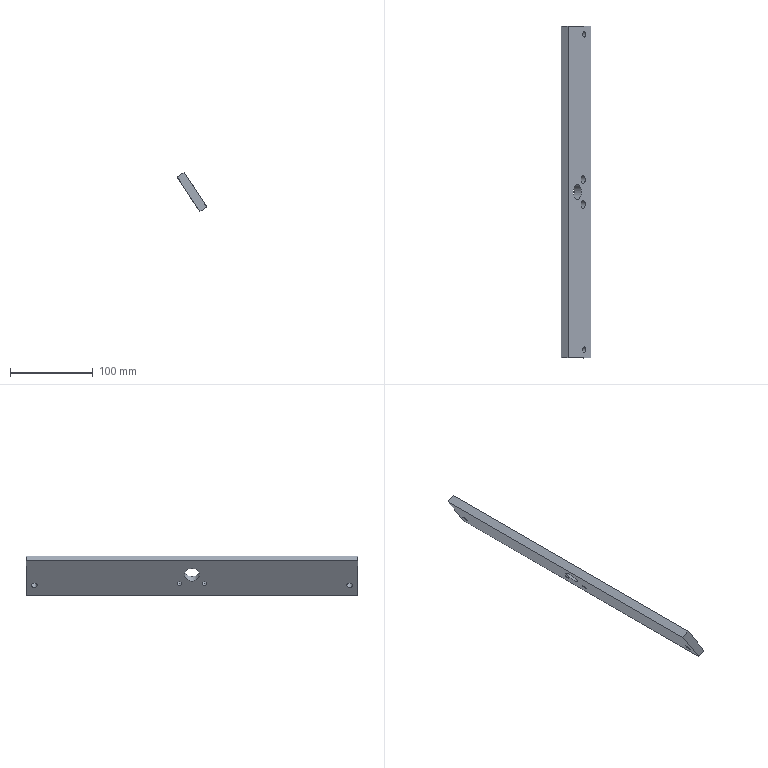Component | SolidWorks | SupportPlate-1 | 1 solid | 22 faces | box 35.72 x 400 x 47.33 mm | volume 195629 mm3 | cylinder 14 | plane 8 | commonest cylinder face diameters 10 x4 5.5 x4 6.8 x4 18 x2
build123d program:
from build123d import *

# Parameters (mm, degrees)
SKETCH1_W                                            = 400
SKETCH1_H                                            = 30
BOSS_EXTRUDE1_DEPTH                                  = 10
M8_TAPPED_HOLE1_D                                    = 6.8
M8_TAPPED_HOLE1_DEPTH                                = 19.75
M8_TAPPED_HOLE1_TIP                                  = 2.043
SKETCH7_W                                            = 400
SKETCH7_H                                            = 10
BOSS_EXTRUDE3_DEPTH                                  = 20
SKETCH9_R                                            = 9
CUT_EXTRUDE2_DEPTH                                   = 204.286
HOLE_SIZE_ACCORDING_TO_THE_TYPE_OF_HEXAG_D           = 5.5
HOLE_SIZE_ACCORDING_TO_THE_TYPE_OF_HEXAG_CBORE_D     = 10
HOLE_SIZE_ACCORDING_TO_THE_TYPE_OF_HEXAG_CBORE_DEPTH = 5.7


with BuildPart() as part:
    # Sketch1 → Boss-Extrude1 (new body)
    with BuildSketch(Plane.XY):
        Rectangle(SKETCH1_W, SKETCH1_H)
    extrude(amount=BOSS_EXTRUDE1_DEPTH)

    # M8 Tapped Hole1
    with Locations(Plane.XY.offset(10)):
        with Locations((-190, 0), (190, 0)):
            Hole(M8_TAPPED_HOLE1_D / 2, depth=M8_TAPPED_HOLE1_DEPTH)
            with Locations((0, 0, -(M8_TAPPED_HOLE1_DEPTH + M8_TAPPED_HOLE1_TIP / 2))):  # 118° drill point
                Cone(0, M8_TAPPED_HOLE1_D / 2, M8_TAPPED_HOLE1_TIP, mode=Mode.SUBTRACT)

    # Sketch7 → Boss-Extrude3 (add)
    with BuildSketch(Plane.XZ.offset(15)):
        with Locations((0, 5)):
            Rectangle(SKETCH7_W, SKETCH7_H)
    extrude(amount=BOSS_EXTRUDE3_DEPTH)

    # Sketch9 → Cut-Extrude2 (cut, through all)
    with BuildSketch(Plane.XY.offset(10)):
        with Locations((0, -15)):
            Circle(SKETCH9_R)
    extrude(amount=-CUT_EXTRUDE2_DEPTH, mode=Mode.SUBTRACT)

    # Hole Size according to the type of hexag (through all)
    with Locations(Plane.XY.offset(10)):
        with Locations((-15, -2.5), (15, -2.5)):
            CounterBoreHole(HOLE_SIZE_ACCORDING_TO_THE_TYPE_OF_HEXAG_D / 2, HOLE_SIZE_ACCORDING_TO_THE_TYPE_OF_HEXAG_CBORE_D / 2, HOLE_SIZE_ACCORDING_TO_THE_TYPE_OF_HEXAG_CBORE_DEPTH)


solid = part.part

# Placed as in the assembly
solid = solid.moved(Location((-212.557, -40.454, -141.988), (0, 56.835, -90)))
STEP:
#1=COLOUR_RGB('',0.7922,0.8196,0.9333);
#2=FILL_AREA_STYLE_COLOUR('',#1);
#3=FILL_AREA_STYLE('',(#2));
#4=SURFACE_STYLE_FILL_AREA(#3);
#5=SURFACE_SIDE_STYLE('',(#4));
#6=SURFACE_STYLE_USAGE(.BOTH.,#5);
#7=PRESENTATION_STYLE_ASSIGNMENT((#6));
#8=CARTESIAN_POINT('',(-8.281,-0.8053,-5.415));
#9=VERTEX_POINT('',#8);
#10=CARTESIAN_POINT('',(-8.281,-1.199,-5.415));
#11=VERTEX_POINT('',#10);
#12=CARTESIAN_POINT('',(-8.281,-1.002,-5.415));
#13=DIRECTION('',(0.8371,-0.,0.5471));
#14=DIRECTION('',(0.,-1.,0.));
#15=AXIS2_PLACEMENT_3D('',#12,#13,#14);
#16=CIRCLE('',#15,0.1969);
#17=EDGE_CURVE('',#9,#11,#16,.T.);
#18=ORIENTED_EDGE('',*,*,#17,.F.);
#19=CARTESIAN_POINT('',(-8.093,-0.8053,-5.292));
#20=VERTEX_POINT('',#19);
#21=CARTESIAN_POINT('',(-8.093,-0.8053,-5.292));
#22=DIRECTION('',(0.8371,-0.,0.5471));
#23=VECTOR('',#22,39.37);
#24=LINE('',#21,#23);
#25=EDGE_CURVE('',#9,#20,#24,.T.);
#26=ORIENTED_EDGE('',*,*,#25,.T.);
#27=CARTESIAN_POINT('',(-8.093,-1.199,-5.292));
#28=VERTEX_POINT('',#27);
#29=CARTESIAN_POINT('',(-8.093,-1.002,-5.292));
#30=DIRECTION('',(0.8371,-0.,0.5471));
#31=DIRECTION('',(0.,-1.,0.));
#32=AXIS2_PLACEMENT_3D('',#29,#30,#31);
#33=CIRCLE('',#32,0.1969);
#34=EDGE_CURVE('',#20,#28,#33,.T.);
#35=ORIENTED_EDGE('',*,*,#34,.T.);
#36=CARTESIAN_POINT('',(-8.093,-1.199,-5.292));
#37=DIRECTION('',(0.8371,-0.,0.5471));
#38=VECTOR('',#37,39.37);
#39=LINE('',#36,#38);
#40=EDGE_CURVE('',#11,#28,#39,.T.);
#41=ORIENTED_EDGE('',*,*,#40,.F.);
#42=EDGE_LOOP('',(#18,#26,#35,#41));
#43=FACE_OUTER_BOUND('',#42,.T.);
#44=CARTESIAN_POINT('',(-8.093,-1.002,-5.292));
#45=DIRECTION('',(0.8371,-0.,0.5471));
#46=DIRECTION('',(0.,-1.,0.));
#47=AXIS2_PLACEMENT_3D('',#44,#45,#46);
#48=CYLINDRICAL_SURFACE('',#47,0.1969);
#49=ADVANCED_FACE('',(#43),#48,.F.);
#50=CARTESIAN_POINT('',(-8.422,-0.8939,-5.508));
#51=VERTEX_POINT('',#50);
#52=CARTESIAN_POINT('',(-8.422,-1.11,-5.508));
#53=VERTEX_POINT('',#52);
#54=CARTESIAN_POINT('',(-8.422,-1.002,-5.508));
#55=DIRECTION('',(0.8371,-0.,0.5471));
#56=DIRECTION('',(0.,-1.,0.));
#57=AXIS2_PLACEMENT_3D('',#54,#55,#56);
#58=CIRCLE('',#57,0.1083);
#59=EDGE_CURVE('',#51,#53,#58,.T.);
#60=ORIENTED_EDGE('',*,*,#59,.F.);
#61=CARTESIAN_POINT('',(-8.281,-0.8939,-5.415));
#62=VERTEX_POINT('',#61);
#63=CARTESIAN_POINT('',(-8.093,-0.8939,-5.292));
#64=DIRECTION('',(0.8371,-0.,0.5471));
#65=VECTOR('',#64,39.37);
#66=LINE('',#63,#65);
#67=EDGE_CURVE('',#51,#62,#66,.T.);
#68=ORIENTED_EDGE('',*,*,#67,.T.);
#69=CARTESIAN_POINT('',(-8.281,-1.11,-5.415));
#70=VERTEX_POINT('',#69);
#71=CARTESIAN_POINT('',(-8.281,-1.002,-5.415));
#72=DIRECTION('',(0.8371,-0.,0.5471));
#73=DIRECTION('',(0.,-1.,0.));
#74=AXIS2_PLACEMENT_3D('',#71,#72,#73);
#75=CIRCLE('',#74,0.1083);
#76=EDGE_CURVE('',#62,#70,#75,.T.);
#77=ORIENTED_EDGE('',*,*,#76,.T.);
#78=CARTESIAN_POINT('',(-8.093,-1.11,-5.292));
#79=DIRECTION('',(0.8371,-0.,0.5471));
#80=VECTOR('',#79,39.37);
#81=LINE('',#78,#80);
#82=EDGE_CURVE('',#53,#70,#81,.T.);
#83=ORIENTED_EDGE('',*,*,#82,.F.);
#84=EDGE_LOOP('',(#60,#68,#77,#83));
#85=FACE_OUTER_BOUND('',#84,.T.);
#86=CARTESIAN_POINT('',(-8.093,-1.002,-5.292));
#87=DIRECTION('',(0.8371,-0.,0.5471));
#88=DIRECTION('',(0.,-1.,0.));
#89=AXIS2_PLACEMENT_3D('',#86,#87,#88);
#90=CYLINDRICAL_SURFACE('',#89,0.1083);
#91=ADVANCED_FACE('',(#85),#90,.F.);
#92=CARTESIAN_POINT('',(-8.281,-1.986,-5.415));
#93=VERTEX_POINT('',#92);
#94=CARTESIAN_POINT('',(-8.281,-2.38,-5.415));
#95=VERTEX_POINT('',#94);
#96=CARTESIAN_POINT('',(-8.281,-2.183,-5.415));
#97=DIRECTION('',(0.8371,-0.,0.5471));
#98=DIRECTION('',(0.,-1.,0.));
#99=AXIS2_PLACEMENT_3D('',#96,#97,#98);
#100=CIRCLE('',#99,0.1969);
#101=EDGE_CURVE('',#93,#95,#100,.T.);
#102=ORIENTED_EDGE('',*,*,#101,.F.);
#103=CARTESIAN_POINT('',(-8.093,-1.986,-5.292));
#104=VERTEX_POINT('',#103);
#105=CARTESIAN_POINT('',(-8.093,-1.986,-5.292));
#106=DIRECTION('',(0.8371,-0.,0.5471));
#107=VECTOR('',#106,39.37);
#108=LINE('',#105,#107);
#109=EDGE_CURVE('',#93,#104,#108,.T.);
#110=ORIENTED_EDGE('',*,*,#109,.T.);
#111=CARTESIAN_POINT('',(-8.093,-2.38,-5.292));
#112=VERTEX_POINT('',#111);
#113=CARTESIAN_POINT('',(-8.093,-2.183,-5.292));
#114=DIRECTION('',(0.8371,-0.,0.5471));
#115=DIRECTION('',(0.,-1.,0.));
#116=AXIS2_PLACEMENT_3D('',#113,#114,#115);
#117=CIRCLE('',#116,0.1969);
#118=EDGE_CURVE('',#104,#112,#117,.T.);
#119=ORIENTED_EDGE('',*,*,#118,.T.);
#120=CARTESIAN_POINT('',(-8.093,-2.38,-5.292));
#121=DIRECTION('',(0.8371,-0.,0.5471));
#122=VECTOR('',#121,39.37);
#123=LINE('',#120,#122);
#124=EDGE_CURVE('',#95,#112,#123,.T.);
#125=ORIENTED_EDGE('',*,*,#124,.F.);
#126=EDGE_LOOP('',(#102,#110,#119,#125));
#127=FACE_OUTER_BOUND('',#126,.T.);
#128=CARTESIAN_POINT('',(-8.093,-2.183,-5.292));
#129=DIRECTION('',(0.8371,-0.,0.5471));
#130=DIRECTION('',(0.,-1.,0.));
#131=AXIS2_PLACEMENT_3D('',#128,#129,#130);
#132=CYLINDRICAL_SURFACE('',#131,0.1969);
#133=ADVANCED_FACE('',(#127),#132,.F.);
#134=CARTESIAN_POINT('',(-8.422,-2.075,-5.508));
#135=VERTEX_POINT('',#134);
#136=CARTESIAN_POINT('',(-8.422,-2.292,-5.508));
#137=VERTEX_POINT('',#136);
#138=CARTESIAN_POINT('',(-8.422,-2.183,-5.508));
#139=DIRECTION('',(0.8371,-0.,0.5471));
#140=DIRECTION('',(0.,-1.,0.));
#141=AXIS2_PLACEMENT_3D('',#138,#139,#140);
#142=CIRCLE('',#141,0.1083);
#143=EDGE_CURVE('',#135,#137,#142,.T.);
#144=ORIENTED_EDGE('',*,*,#143,.F.);
#145=CARTESIAN_POINT('',(-8.281,-2.075,-5.415));
#146=VERTEX_POINT('',#145);
#147=CARTESIAN_POINT('',(-8.093,-2.075,-5.292));
#148=DIRECTION('',(0.8371,-0.,0.5471));
#149=VECTOR('',#148,39.37);
#150=LINE('',#147,#149);
#151=EDGE_CURVE('',#135,#146,#150,.T.);
#152=ORIENTED_EDGE('',*,*,#151,.T.);
#153=CARTESIAN_POINT('',(-8.281,-2.292,-5.415));
#154=VERTEX_POINT('',#153);
#155=CARTESIAN_POINT('',(-8.281,-2.183,-5.415));
#156=DIRECTION('',(0.8371,-0.,0.5471));
#157=DIRECTION('',(0.,-1.,0.));
#158=AXIS2_PLACEMENT_3D('',#155,#156,#157);
#159=CIRCLE('',#158,0.1083);
#160=EDGE_CURVE('',#146,#154,#159,.T.);
#161=ORIENTED_EDGE('',*,*,#160,.T.);
#162=CARTESIAN_POINT('',(-8.093,-2.292,-5.292));
#163=DIRECTION('',(0.8371,-0.,0.5471));
#164=VECTOR('',#163,39.37);
#165=LINE('',#162,#164);
#166=EDGE_CURVE('',#137,#154,#165,.T.);
#167=ORIENTED_EDGE('',*,*,#166,.F.);
#168=EDGE_LOOP('',(#144,#152,#161,#167));
#169=FACE_OUTER_BOUND('',#168,.T.);
#170=CARTESIAN_POINT('',(-8.093,-2.183,-5.292));
#171=DIRECTION('',(0.8371,-0.,0.5471));
#172=DIRECTION('',(0.,-1.,0.));
#173=AXIS2_PLACEMENT_3D('',#170,#171,#172);
#174=CYLINDRICAL_SURFACE('',#173,0.1083);
#175=ADVANCED_FACE('',(#169),#174,.F.);
#176=CARTESIAN_POINT('',(-8.691,-1.238,-5.096));
#177=VERTEX_POINT('',#176);
#178=CARTESIAN_POINT('',(-8.691,-1.947,-5.096));
#179=VERTEX_POINT('',#178);
#180=CARTESIAN_POINT('',(-8.691,-1.593,-5.096));
#181=DIRECTION('',(0.8371,-0.,0.5471));
#182=DIRECTION('',(0.,-1.,0.));
#183=AXIS2_PLACEMENT_3D('',#180,#181,#182);
#184=CIRCLE('',#183,0.3543);
#185=EDGE_CURVE('',#177,#179,#184,.T.);
#186=ORIENTED_EDGE('',*,*,#185,.F.);
#187=CARTESIAN_POINT('',(-8.362,-1.238,-4.88));
#188=VERTEX_POINT('',#187);
#189=CARTESIAN_POINT('',(-8.691,-1.238,-5.096));
#190=DIRECTION('',(0.8371,-0.,0.5471));
#191=VECTOR('',#190,39.37);
#192=LINE('',#189,#191);
#193=EDGE_CURVE('',#177,#188,#192,.T.);
#194=ORIENTED_EDGE('',*,*,#193,.T.);
#195=CARTESIAN_POINT('',(-8.362,-1.947,-4.88));
#196=VERTEX_POINT('',#195);
#197=CARTESIAN_POINT('',(-8.362,-1.593,-4.88));
#198=DIRECTION('',(0.8371,-0.,0.5471));
#199=DIRECTION('',(0.,-1.,0.));
#200=AXIS2_PLACEMENT_3D('',#197,#198,#199);
#201=CIRCLE('',#200,0.3543);
#202=EDGE_CURVE('',#188,#196,#201,.T.);
#203=ORIENTED_EDGE('',*,*,#202,.T.);
#204=CARTESIAN_POINT('',(-8.691,-1.947,-5.096));
#205=DIRECTION('',(0.8371,-0.,0.5471));
#206=VECTOR('',#205,39.37);
#207=LINE('',#204,#206);
#208=EDGE_CURVE('',#179,#196,#207,.T.);
#209=ORIENTED_EDGE('',*,*,#208,.F.);
#210=EDGE_LOOP('',(#186,#194,#203,#209));
#211=FACE_OUTER_BOUND('',#210,.T.);
#212=CARTESIAN_POINT('',(-8.691,-1.593,-5.096));
#213=DIRECTION('',(0.8371,-0.,0.5471));
#214=DIRECTION('',(0.,-1.,0.));
#215=AXIS2_PLACEMENT_3D('',#212,#213,#214);
#216=CYLINDRICAL_SURFACE('',#215,0.3543);
#217=ADVANCED_FACE('',(#211),#216,.F.);
#218=CARTESIAN_POINT('',(-8.368,5.754,-5.59));
#219=VERTEX_POINT('',#218);
#220=CARTESIAN_POINT('',(-8.368,6.021,-5.59));
#221=VERTEX_POINT('',#220);
#222=CARTESIAN_POINT('',(-8.368,5.888,-5.59));
#223=DIRECTION('',(-0.8371,0.,-0.5471));
#224=DIRECTION('',(0.,1.,0.));
#225=AXIS2_PLACEMENT_3D('',#222,#223,#224);
#226=CIRCLE('',#225,0.1339);
#227=EDGE_CURVE('',#219,#221,#226,.T.);
#228=ORIENTED_EDGE('',*,*,#227,.T.);
#229=CARTESIAN_POINT('',(-8.039,6.021,-5.375));
#230=VERTEX_POINT('',#229);
#231=CARTESIAN_POINT('',(-8.039,6.021,-5.375));
#232=DIRECTION('',(0.8371,-0.,0.5471));
#233=VECTOR('',#232,39.37);
#234=LINE('',#231,#233);
#235=EDGE_CURVE('',#221,#230,#234,.T.);
#236=ORIENTED_EDGE('',*,*,#235,.T.);
#237=CARTESIAN_POINT('',(-8.039,5.754,-5.375));
#238=VERTEX_POINT('',#237);
#239=CARTESIAN_POINT('',(-8.039,5.888,-5.375));
#240=DIRECTION('',(0.8371,-0.,0.5471));
#241=DIRECTION('',(0.,-1.,0.));
#242=AXIS2_PLACEMENT_3D('',#239,#240,#241);
#243=CIRCLE('',#242,0.1339);
#244=EDGE_CURVE('',#230,#238,#243,.T.);
#245=ORIENTED_EDGE('',*,*,#244,.T.);
#246=CARTESIAN_POINT('',(-8.039,5.754,-5.375));
#247=DIRECTION('',(0.8371,-0.,0.5471));
#248=VECTOR('',#247,39.37);
#249=LINE('',#246,#248);
#250=EDGE_CURVE('',#219,#238,#249,.T.);
#251=ORIENTED_EDGE('',*,*,#250,.F.);
#252=EDGE_LOOP('',(#228,#236,#245,#251));
#253=FACE_OUTER_BOUND('',#252,.T.);
#254=CARTESIAN_POINT('',(-8.039,5.888,-5.375));
#255=DIRECTION('',(0.8371,-0.,0.5471));
#256=DIRECTION('',(0.,-1.,0.));
#257=AXIS2_PLACEMENT_3D('',#254,#255,#256);
#258=CYLINDRICAL_SURFACE('',#257,0.1339);
#259=ADVANCED_FACE('',(#253),#258,.F.);
#260=CARTESIAN_POINT('',(-8.368,-9.207,-5.59));
#261=VERTEX_POINT('',#260);
#262=CARTESIAN_POINT('',(-8.368,-8.939,-5.59));
#263=VERTEX_POINT('',#262);
#264=CARTESIAN_POINT('',(-8.368,-9.073,-5.59));
#265=DIRECTION('',(-0.8371,0.,-0.5471));
#266=DIRECTION('',(0.,1.,0.));
#267=AXIS2_PLACEMENT_3D('',#264,#265,#266);
#268=CIRCLE('',#267,0.1339);
#269=EDGE_CURVE('',#261,#263,#268,.T.);
#270=ORIENTED_EDGE('',*,*,#269,.T.);
#271=CARTESIAN_POINT('',(-8.039,-8.939,-5.375));
#272=VERTEX_POINT('',#271);
#273=CARTESIAN_POINT('',(-8.039,-8.939,-5.375));
#274=DIRECTION('',(0.8371,-0.,0.5471));
#275=VECTOR('',#274,39.37);
#276=LINE('',#273,#275);
#277=EDGE_CURVE('',#263,#272,#276,.T.);
#278=ORIENTED_EDGE('',*,*,#277,.T.);
#279=CARTESIAN_POINT('',(-8.039,-9.207,-5.375));
#280=VERTEX_POINT('',#279);
#281=CARTESIAN_POINT('',(-8.039,-9.073,-5.375));
#282=DIRECTION('',(0.8371,-0.,0.5471));
#283=DIRECTION('',(0.,-1.,0.));
#284=AXIS2_PLACEMENT_3D('',#281,#282,#283);
#285=CIRCLE('',#284,0.1339);
#286=EDGE_CURVE('',#272,#280,#285,.T.);
#287=ORIENTED_EDGE('',*,*,#286,.T.);
#288=CARTESIAN_POINT('',(-8.039,-9.207,-5.375));
#289=DIRECTION('',(0.8371,-0.,0.5471));
#290=VECTOR('',#289,39.37);
#291=LINE('',#288,#290);
#292=EDGE_CURVE('',#261,#280,#291,.T.);
#293=ORIENTED_EDGE('',*,*,#292,.F.);
#294=EDGE_LOOP('',(#270,#278,#287,#293));
#295=FACE_OUTER_BOUND('',#294,.T.);
#296=CARTESIAN_POINT('',(-8.039,-9.073,-5.375));
#297=DIRECTION('',(0.8371,-0.,0.5471));
#298=DIRECTION('',(0.,-1.,0.));
#299=AXIS2_PLACEMENT_3D('',#296,#297,#298);
#300=CYLINDRICAL_SURFACE('',#299,0.1339);
#301=ADVANCED_FACE('',(#295),#300,.F.);
#302=CARTESIAN_POINT('',(-9.122,-9.467,-4.437));
#303=VERTEX_POINT('',#302);
#304=CARTESIAN_POINT('',(-8.045,-9.467,-6.084));
#305=VERTEX_POINT('',#304);
#306=CARTESIAN_POINT('',(-8.691,-9.467,-5.096));
#307=DIRECTION('',(0.5471,-0.,-0.8371));
#308=VECTOR('',#307,39.37);
#309=LINE('',#306,#308);
#310=EDGE_CURVE('',#303,#305,#309,.T.);
#311=ORIENTED_EDGE('',*,*,#310,.T.);
#312=CARTESIAN_POINT('',(-7.716,-9.467,-5.869));
#313=VERTEX_POINT('',#312);
#314=CARTESIAN_POINT('',(-7.716,-9.467,-5.869));
#315=DIRECTION('',(-0.8371,0.,-0.5471));
#316=VECTOR('',#315,39.37);
#317=LINE('',#314,#316);
#318=EDGE_CURVE('',#313,#305,#317,.T.);
#319=ORIENTED_EDGE('',*,*,#318,.F.);
#320=CARTESIAN_POINT('',(-8.793,-9.467,-4.221));
#321=VERTEX_POINT('',#320);
#322=CARTESIAN_POINT('',(-8.362,-9.467,-4.88));
#323=DIRECTION('',(0.5471,-0.,-0.8371));
#324=VECTOR('',#323,39.37);
#325=LINE('',#322,#324);
#326=EDGE_CURVE('',#321,#313,#325,.T.);
#327=ORIENTED_EDGE('',*,*,#326,.F.);
#328=CARTESIAN_POINT('',(-8.793,-9.467,-4.221));
#329=DIRECTION('',(0.8371,-0.,0.5471));
#330=VECTOR('',#329,39.37);
#331=LINE('',#328,#330);
#332=EDGE_CURVE('',#303,#321,#331,.T.);
#333=ORIENTED_EDGE('',*,*,#332,.F.);
#334=EDGE_LOOP('',(#311,#319,#327,#333));
#335=FACE_OUTER_BOUND('',#334,.T.);
#336=CARTESIAN_POINT('',(-8.362,-9.467,-4.88));
#337=DIRECTION('',(0.,1.,-0.));
#338=DIRECTION('',(0.8371,-0.,0.5471));
#339=AXIS2_PLACEMENT_3D('',#336,#337,#338);
#340=PLANE('',#339);
#341=ADVANCED_FACE('',(#335),#340,.F.);
#342=CARTESIAN_POINT('',(-8.045,6.281,-6.084));
#343=VERTEX_POINT('',#342);
#344=CARTESIAN_POINT('',(-8.045,6.281,-6.084));
#345=DIRECTION('',(0.,1.,-0.));
#346=VECTOR('',#345,39.37);
#347=LINE('',#344,#346);
#348=EDGE_CURVE('',#305,#343,#347,.T.);
#349=ORIENTED_EDGE('',*,*,#348,.T.);
#350=CARTESIAN_POINT('',(-7.716,6.281,-5.869));
#351=VERTEX_POINT('',#350);
#352=CARTESIAN_POINT('',(-7.716,6.281,-5.869));
#353=DIRECTION('',(-0.8371,0.,-0.5471));
#354=VECTOR('',#353,39.37);
#355=LINE('',#352,#354);
#356=EDGE_CURVE('',#351,#343,#355,.T.);
#357=ORIENTED_EDGE('',*,*,#356,.F.);
#358=CARTESIAN_POINT('',(-7.716,6.281,-5.869));
#359=DIRECTION('',(0.,1.,-0.));
#360=VECTOR('',#359,39.37);
#361=LINE('',#358,#360);
#362=EDGE_CURVE('',#313,#351,#361,.T.);
#363=ORIENTED_EDGE('',*,*,#362,.F.);
#364=ORIENTED_EDGE('',*,*,#318,.T.);
#365=EDGE_LOOP('',(#349,#357,#363,#364));
#366=FACE_OUTER_BOUND('',#365,.T.);
#367=CARTESIAN_POINT('',(-7.716,6.281,-5.869));
#368=DIRECTION('',(-0.5471,0.,0.8371));
#369=DIRECTION('',(-0.8371,0.,-0.5471));
#370=AXIS2_PLACEMENT_3D('',#367,#368,#369);
#371=PLANE('',#370);
#372=ADVANCED_FACE('',(#366),#371,.F.);
#373=CARTESIAN_POINT('',(-9.122,6.281,-4.437));
#374=VERTEX_POINT('',#373);
#375=CARTESIAN_POINT('',(-8.691,6.281,-5.096));
#376=DIRECTION('',(-0.5471,0.,0.8371));
#377=VECTOR('',#376,39.37);
#378=LINE('',#375,#377);
#379=EDGE_CURVE('',#343,#374,#378,.T.);
#380=ORIENTED_EDGE('',*,*,#379,.T.);
#381=CARTESIAN_POINT('',(-8.793,6.281,-4.221));
#382=VERTEX_POINT('',#381);
#383=CARTESIAN_POINT('',(-8.793,6.281,-4.221));
#384=DIRECTION('',(-0.8371,0.,-0.5471));
#385=VECTOR('',#384,39.37);
#386=LINE('',#383,#385);
#387=EDGE_CURVE('',#382,#374,#386,.T.);
#388=ORIENTED_EDGE('',*,*,#387,.F.);
#389=CARTESIAN_POINT('',(-8.362,6.281,-4.88));
#390=DIRECTION('',(-0.5471,0.,0.8371));
#391=VECTOR('',#390,39.37);
#392=LINE('',#389,#391);
#393=EDGE_CURVE('',#351,#382,#392,.T.);
#394=ORIENTED_EDGE('',*,*,#393,.F.);
#395=ORIENTED_EDGE('',*,*,#356,.T.);
#396=EDGE_LOOP('',(#380,#388,#394,#395));
#397=FACE_OUTER_BOUND('',#396,.T.);
#398=CARTESIAN_POINT('',(-8.362,6.281,-4.88));
#399=DIRECTION('',(-0.,-1.,0.));
#400=DIRECTION('',(-0.8371,0.,-0.5471));
#401=AXIS2_PLACEMENT_3D('',#398,#399,#400);
#402=PLANE('',#401);
#403=ADVANCED_FACE('',(#397),#402,.F.);
#404=CARTESIAN_POINT('',(-8.093,-1.002,-5.292));
#405=DIRECTION('',(0.8371,-0.,0.5471));
#406=DIRECTION('',(0.,-1.,0.));
#407=AXIS2_PLACEMENT_3D('',#404,#405,#406);
#408=CIRCLE('',#407,0.1969);
#409=EDGE_CURVE('',#28,#20,#408,.T.);
#410=ORIENTED_EDGE('',*,*,#409,.F.);
#411=ORIENTED_EDGE('',*,*,#34,.F.);
#412=EDGE_LOOP('',(#410,#411));
#413=FACE_BOUND('',#412,.T.);
#414=CARTESIAN_POINT('',(-8.093,-2.183,-5.292));
#415=DIRECTION('',(0.8371,-0.,0.5471));
#416=DIRECTION('',(0.,-1.,0.));
#417=AXIS2_PLACEMENT_3D('',#414,#415,#416);
#418=CIRCLE('',#417,0.1969);
#419=EDGE_CURVE('',#112,#104,#418,.T.);
#420=ORIENTED_EDGE('',*,*,#419,.F.);
#421=ORIENTED_EDGE('',*,*,#118,.F.);
#422=EDGE_LOOP('',(#420,#421));
#423=FACE_BOUND('',#422,.T.);
#424=CARTESIAN_POINT('',(-8.362,-1.593,-4.88));
#425=DIRECTION('',(0.8371,-0.,0.5471));
#426=DIRECTION('',(0.,-1.,0.));
#427=AXIS2_PLACEMENT_3D('',#424,#425,#426);
#428=CIRCLE('',#427,0.3543);
#429=EDGE_CURVE('',#196,#188,#428,.T.);
#430=ORIENTED_EDGE('',*,*,#429,.F.);
#431=ORIENTED_EDGE('',*,*,#202,.F.);
#432=EDGE_LOOP('',(#430,#431));
#433=FACE_BOUND('',#432,.T.);
#434=CARTESIAN_POINT('',(-8.039,5.888,-5.375));
#435=DIRECTION('',(0.8371,-0.,0.5471));
#436=DIRECTION('',(0.,-1.,0.));
#437=AXIS2_PLACEMENT_3D('',#434,#435,#436);
#438=CIRCLE('',#437,0.1339);
#439=EDGE_CURVE('',#238,#230,#438,.T.);
#440=ORIENTED_EDGE('',*,*,#439,.F.);
#441=ORIENTED_EDGE('',*,*,#244,.F.);
#442=EDGE_LOOP('',(#440,#441));
#443=FACE_BOUND('',#442,.T.);
#444=CARTESIAN_POINT('',(-8.039,-9.073,-5.375));
#445=DIRECTION('',(0.8371,-0.,0.5471));
#446=DIRECTION('',(0.,-1.,0.));
#447=AXIS2_PLACEMENT_3D('',#444,#445,#446);
#448=CIRCLE('',#447,0.1339);
#449=EDGE_CURVE('',#280,#272,#448,.T.);
#450=ORIENTED_EDGE('',*,*,#449,.F.);
#451=ORIENTED_EDGE('',*,*,#286,.F.);
#452=EDGE_LOOP('',(#450,#451));
#453=FACE_BOUND('',#452,.T.);
#454=ORIENTED_EDGE('',*,*,#326,.T.);
#455=ORIENTED_EDGE('',*,*,#362,.T.);
#456=ORIENTED_EDGE('',*,*,#393,.T.);
#457=CARTESIAN_POINT('',(-8.793,6.281,-4.221));
#458=DIRECTION('',(0.,1.,-0.));
#459=VECTOR('',#458,39.37);
#460=LINE('',#457,#459);
#461=EDGE_CURVE('',#321,#382,#460,.T.);
#462=ORIENTED_EDGE('',*,*,#461,.F.);
#463=EDGE_LOOP('',(#454,#455,#456,#462));
#464=FACE_OUTER_BOUND('',#463,.T.);
#465=CARTESIAN_POINT('',(-8.039,-1.593,-5.375));
#466=DIRECTION('',(-0.8371,0.,-0.5471));
#467=DIRECTION('',(0.,1.,-0.));
#468=AXIS2_PLACEMENT_3D('',#465,#466,#467);
#469=PLANE('',#468);
#470=ADVANCED_FACE('',(#413,#423,#433,#443,#453,#464),#469,.F.);
#471=CARTESIAN_POINT('',(-8.422,-1.002,-5.508));
#472=DIRECTION('',(0.8371,-0.,0.5471));
#473=DIRECTION('',(0.,-1.,0.));
#474=AXIS2_PLACEMENT_3D('',#471,#472,#473);
#475=CIRCLE('',#474,0.1083);
#476=EDGE_CURVE('',#53,#51,#475,.T.);
#477=ORIENTED_EDGE('',*,*,#476,.T.);
#478=ORIENTED_EDGE('',*,*,#59,.T.);
#479=EDGE_LOOP('',(#477,#478));
#480=FACE_BOUND('',#479,.T.);
#481=CARTESIAN_POINT('',(-8.422,-2.183,-5.508));
#482=DIRECTION('',(0.8371,-0.,0.5471));
#483=DIRECTION('',(0.,-1.,0.));
#484=AXIS2_PLACEMENT_3D('',#481,#482,#483);
#485=CIRCLE('',#484,0.1083);
#486=EDGE_CURVE('',#137,#135,#485,.T.);
#487=ORIENTED_EDGE('',*,*,#486,.T.);
#488=ORIENTED_EDGE('',*,*,#143,.T.);
#489=EDGE_LOOP('',(#487,#488));
#490=FACE_BOUND('',#489,.T.);
#491=CARTESIAN_POINT('',(-8.691,-1.593,-5.096));
#492=DIRECTION('',(0.8371,-0.,0.5471));
#493=DIRECTION('',(0.,-1.,0.));
#494=AXIS2_PLACEMENT_3D('',#491,#492,#493);
#495=CIRCLE('',#494,0.3543);
#496=EDGE_CURVE('',#179,#177,#495,.T.);
#497=ORIENTED_EDGE('',*,*,#496,.T.);
#498=ORIENTED_EDGE('',*,*,#185,.T.);
#499=EDGE_LOOP('',(#497,#498));
#500=FACE_BOUND('',#499,.T.);
#501=ORIENTED_EDGE('',*,*,#227,.F.);
#502=CARTESIAN_POINT('',(-8.368,5.888,-5.59));
#503=DIRECTION('',(-0.8371,0.,-0.5471));
#504=DIRECTION('',(0.,1.,0.));
#505=AXIS2_PLACEMENT_3D('',#502,#503,#504);
#506=CIRCLE('',#505,0.1339);
#507=EDGE_CURVE('',#221,#219,#506,.T.);
#508=ORIENTED_EDGE('',*,*,#507,.F.);
#509=EDGE_LOOP('',(#501,#508));
#510=FACE_BOUND('',#509,.T.);
#511=ORIENTED_EDGE('',*,*,#269,.F.);
#512=CARTESIAN_POINT('',(-8.368,-9.073,-5.59));
#513=DIRECTION('',(-0.8371,0.,-0.5471));
#514=DIRECTION('',(0.,1.,0.));
#515=AXIS2_PLACEMENT_3D('',#512,#513,#514);
#516=CIRCLE('',#515,0.1339);
#517=EDGE_CURVE('',#263,#261,#516,.T.);
#518=ORIENTED_EDGE('',*,*,#517,.F.);
#519=EDGE_LOOP('',(#511,#518));
#520=FACE_BOUND('',#519,.T.);
#521=ORIENTED_EDGE('',*,*,#310,.F.);
#522=CARTESIAN_POINT('',(-9.122,6.281,-4.437));
#523=DIRECTION('',(-0.,-1.,0.));
#524=VECTOR('',#523,39.37);
#525=LINE('',#522,#524);
#526=EDGE_CURVE('',#374,#303,#525,.T.);
#527=ORIENTED_EDGE('',*,*,#526,.F.);
#528=ORIENTED_EDGE('',*,*,#379,.F.);
#529=ORIENTED_EDGE('',*,*,#348,.F.);
#530=EDGE_LOOP('',(#521,#527,#528,#529));
#531=FACE_OUTER_BOUND('',#530,.T.);
#532=CARTESIAN_POINT('',(-8.368,-1.593,-5.59));
#533=DIRECTION('',(-0.8371,0.,-0.5471));
#534=DIRECTION('',(0.,1.,-0.));
#535=AXIS2_PLACEMENT_3D('',#532,#533,#534);
#536=PLANE('',#535);
#537=ADVANCED_FACE('',(#480,#490,#500,#510,#520,#531),#536,.T.);
#538=ORIENTED_EDGE('',*,*,#277,.F.);
#539=ORIENTED_EDGE('',*,*,#517,.T.);
#540=ORIENTED_EDGE('',*,*,#292,.T.);
#541=ORIENTED_EDGE('',*,*,#449,.T.);
#542=EDGE_LOOP('',(#538,#539,#540,#541));
#543=FACE_OUTER_BOUND('',#542,.T.);
#544=CARTESIAN_POINT('',(-8.039,-9.073,-5.375));
#545=DIRECTION('',(0.8371,-0.,0.5471));
#546=DIRECTION('',(0.,-1.,0.));
#547=AXIS2_PLACEMENT_3D('',#544,#545,#546);
#548=CYLINDRICAL_SURFACE('',#547,0.1339);
#549=ADVANCED_FACE('',(#543),#548,.F.);
#550=ORIENTED_EDGE('',*,*,#235,.F.);
#551=ORIENTED_EDGE('',*,*,#507,.T.);
#552=ORIENTED_EDGE('',*,*,#250,.T.);
#553=ORIENTED_EDGE('',*,*,#439,.T.);
#554=EDGE_LOOP('',(#550,#551,#552,#553));
#555=FACE_OUTER_BOUND('',#554,.T.);
#556=CARTESIAN_POINT('',(-8.039,5.888,-5.375));
#557=DIRECTION('',(0.8371,-0.,0.5471));
#558=DIRECTION('',(0.,-1.,0.));
#559=AXIS2_PLACEMENT_3D('',#556,#557,#558);
#560=CYLINDRICAL_SURFACE('',#559,0.1339);
#561=ADVANCED_FACE('',(#555),#560,.F.);
#562=ORIENTED_EDGE('',*,*,#387,.T.);
#563=ORIENTED_EDGE('',*,*,#526,.T.);
#564=ORIENTED_EDGE('',*,*,#332,.T.);
#565=ORIENTED_EDGE('',*,*,#461,.T.);
#566=EDGE_LOOP('',(#562,#563,#564,#565));
#567=FACE_OUTER_BOUND('',#566,.T.);
#568=CARTESIAN_POINT('',(-9.122,-1.593,-4.437));
#569=DIRECTION('',(-0.5471,0.,0.8371));
#570=DIRECTION('',(-0.8371,0.,-0.5471));
#571=AXIS2_PLACEMENT_3D('',#568,#569,#570);
#572=PLANE('',#571);
#573=ADVANCED_FACE('',(#567),#572,.T.);
#574=ORIENTED_EDGE('',*,*,#193,.F.);
#575=ORIENTED_EDGE('',*,*,#496,.F.);
#576=ORIENTED_EDGE('',*,*,#208,.T.);
#577=ORIENTED_EDGE('',*,*,#429,.T.);
#578=EDGE_LOOP('',(#574,#575,#576,#577));
#579=FACE_OUTER_BOUND('',#578,.T.);
#580=CARTESIAN_POINT('',(-8.691,-1.593,-5.096));
#581=DIRECTION('',(0.8371,-0.,0.5471));
#582=DIRECTION('',(0.,-1.,0.));
#583=AXIS2_PLACEMENT_3D('',#580,#581,#582);
#584=CYLINDRICAL_SURFACE('',#583,0.3543);
#585=ADVANCED_FACE('',(#579),#584,.F.);
#586=ORIENTED_EDGE('',*,*,#151,.F.);
#587=ORIENTED_EDGE('',*,*,#486,.F.);
#588=ORIENTED_EDGE('',*,*,#166,.T.);
#589=CARTESIAN_POINT('',(-8.281,-2.183,-5.415));
#590=DIRECTION('',(0.8371,-0.,0.5471));
#591=DIRECTION('',(0.,-1.,0.));
#592=AXIS2_PLACEMENT_3D('',#589,#590,#591);
#593=CIRCLE('',#592,0.1083);
#594=EDGE_CURVE('',#154,#146,#593,.T.);
#595=ORIENTED_EDGE('',*,*,#594,.T.);
#596=EDGE_LOOP('',(#586,#587,#588,#595));
#597=FACE_OUTER_BOUND('',#596,.T.);
#598=CARTESIAN_POINT('',(-8.093,-2.183,-5.292));
#599=DIRECTION('',(0.8371,-0.,0.5471));
#600=DIRECTION('',(0.,-1.,0.));
#601=AXIS2_PLACEMENT_3D('',#598,#599,#600);
#602=CYLINDRICAL_SURFACE('',#601,0.1083);
#603=ADVANCED_FACE('',(#597),#602,.F.);
#604=ORIENTED_EDGE('',*,*,#594,.F.);
#605=ORIENTED_EDGE('',*,*,#160,.F.);
#606=EDGE_LOOP('',(#604,#605));
#607=FACE_BOUND('',#606,.T.);
#608=CARTESIAN_POINT('',(-8.281,-2.183,-5.415));
#609=DIRECTION('',(0.8371,-0.,0.5471));
#610=DIRECTION('',(0.,-1.,0.));
#611=AXIS2_PLACEMENT_3D('',#608,#609,#610);
#612=CIRCLE('',#611,0.1969);
#613=EDGE_CURVE('',#95,#93,#612,.T.);
#614=ORIENTED_EDGE('',*,*,#613,.T.);
#615=ORIENTED_EDGE('',*,*,#101,.T.);
#616=EDGE_LOOP('',(#614,#615));
#617=FACE_OUTER_BOUND('',#616,.T.);
#618=CARTESIAN_POINT('',(-8.281,-2.292,-5.415));
#619=DIRECTION('',(-0.8371,0.,-0.5471));
#620=DIRECTION('',(0.,1.,-0.));
#621=AXIS2_PLACEMENT_3D('',#618,#619,#620);
#622=PLANE('',#621);
#623=ADVANCED_FACE('',(#607,#617),#622,.F.);
#624=ORIENTED_EDGE('',*,*,#109,.F.);
#625=ORIENTED_EDGE('',*,*,#613,.F.);
#626=ORIENTED_EDGE('',*,*,#124,.T.);
#627=ORIENTED_EDGE('',*,*,#419,.T.);
#628=EDGE_LOOP('',(#624,#625,#626,#627));
#629=FACE_OUTER_BOUND('',#628,.T.);
#630=CARTESIAN_POINT('',(-8.093,-2.183,-5.292));
#631=DIRECTION('',(0.8371,-0.,0.5471));
#632=DIRECTION('',(0.,-1.,0.));
#633=AXIS2_PLACEMENT_3D('',#630,#631,#632);
#634=CYLINDRICAL_SURFACE('',#633,0.1969);
#635=ADVANCED_FACE('',(#629),#634,.F.);
#636=ORIENTED_EDGE('',*,*,#67,.F.);
#637=ORIENTED_EDGE('',*,*,#476,.F.);
#638=ORIENTED_EDGE('',*,*,#82,.T.);
#639=CARTESIAN_POINT('',(-8.281,-1.002,-5.415));
#640=DIRECTION('',(0.8371,-0.,0.5471));
#641=DIRECTION('',(0.,-1.,0.));
#642=AXIS2_PLACEMENT_3D('',#639,#640,#641);
#643=CIRCLE('',#642,0.1083);
#644=EDGE_CURVE('',#70,#62,#643,.T.);
#645=ORIENTED_EDGE('',*,*,#644,.T.);
#646=EDGE_LOOP('',(#636,#637,#638,#645));
#647=FACE_OUTER_BOUND('',#646,.T.);
#648=CARTESIAN_POINT('',(-8.093,-1.002,-5.292));
#649=DIRECTION('',(0.8371,-0.,0.5471));
#650=DIRECTION('',(0.,-1.,0.));
#651=AXIS2_PLACEMENT_3D('',#648,#649,#650);
#652=CYLINDRICAL_SURFACE('',#651,0.1083);
#653=ADVANCED_FACE('',(#647),#652,.F.);
#654=ORIENTED_EDGE('',*,*,#644,.F.);
#655=ORIENTED_EDGE('',*,*,#76,.F.);
#656=EDGE_LOOP('',(#654,#655));
#657=FACE_BOUND('',#656,.T.);
#658=CARTESIAN_POINT('',(-8.281,-1.002,-5.415));
#659=DIRECTION('',(0.8371,-0.,0.5471));
#660=DIRECTION('',(0.,-1.,0.));
#661=AXIS2_PLACEMENT_3D('',#658,#659,#660);
#662=CIRCLE('',#661,0.1969);
#663=EDGE_CURVE('',#11,#9,#662,.T.);
#664=ORIENTED_EDGE('',*,*,#663,.T.);
#665=ORIENTED_EDGE('',*,*,#17,.T.);
#666=EDGE_LOOP('',(#664,#665));
#667=FACE_OUTER_BOUND('',#666,.T.);
#668=CARTESIAN_POINT('',(-8.281,-1.11,-5.415));
#669=DIRECTION('',(-0.8371,0.,-0.5471));
#670=DIRECTION('',(0.,1.,-0.));
#671=AXIS2_PLACEMENT_3D('',#668,#669,#670);
#672=PLANE('',#671);
#673=ADVANCED_FACE('',(#657,#667),#672,.F.);
#674=ORIENTED_EDGE('',*,*,#25,.F.);
#675=ORIENTED_EDGE('',*,*,#663,.F.);
#676=ORIENTED_EDGE('',*,*,#40,.T.);
#677=ORIENTED_EDGE('',*,*,#409,.T.);
#678=EDGE_LOOP('',(#674,#675,#676,#677));
#679=FACE_OUTER_BOUND('',#678,.T.);
#680=CARTESIAN_POINT('',(-8.093,-1.002,-5.292));
#681=DIRECTION('',(0.8371,-0.,0.5471));
#682=DIRECTION('',(0.,-1.,0.));
#683=AXIS2_PLACEMENT_3D('',#680,#681,#682);
#684=CYLINDRICAL_SURFACE('',#683,0.1969);
#685=ADVANCED_FACE('',(#679),#684,.F.);
#686=CLOSED_SHELL('',(#49,#91,#133,#175,#217,#259,#301,#341,#372,#403,#470,#537,#549,#561,#573,#585,#603,#623,#635,#653,#673,#685));
#687=MANIFOLD_SOLID_BREP('',#686);
#688=STYLED_ITEM('',(#7),#687);
#689=(LENGTH_UNIT()NAMED_UNIT(*)SI_UNIT($,.METRE.));
#690=LENGTH_MEASURE_WITH_UNIT(LENGTH_MEASURE(0.0254),#689);
#691=DIMENSIONAL_EXPONENTS(1.,0.,0.,0.,0.,0.,0.);
#692=(CONVERSION_BASED_UNIT('',#690)LENGTH_UNIT()NAMED_UNIT(#691));
#693=UNCERTAINTY_MEASURE_WITH_UNIT(LENGTH_MEASURE(0.00001),#692,'','');
#694=(NAMED_UNIT(*)PLANE_ANGLE_UNIT()SI_UNIT($,.RADIAN.));
#695=(NAMED_UNIT(*)SI_UNIT($,.STERADIAN.)SOLID_ANGLE_UNIT());
#696=(GEOMETRIC_REPRESENTATION_CONTEXT(3)GLOBAL_UNCERTAINTY_ASSIGNED_CONTEXT((#693))GLOBAL_UNIT_ASSIGNED_CONTEXT((#692,#694,#695))REPRESENTATION_CONTEXT('',''));
#697=MECHANICAL_DESIGN_GEOMETRIC_PRESENTATION_REPRESENTATION('',(#688),#696);
#698=PRESENTATION_LAYER_ASSIGNMENT('','',(#688));
#699=CARTESIAN_POINT('',(0.,0.,0.));
#700=DIRECTION('',(0.,0.,1.));
#701=DIRECTION('',(1.,0.,0.));
#702=AXIS2_PLACEMENT_3D('',#699,#700,#701);
#703=(LENGTH_UNIT()NAMED_UNIT(*)SI_UNIT($,.METRE.));
#704=LENGTH_MEASURE_WITH_UNIT(LENGTH_MEASURE(0.0254),#703);
#705=DIMENSIONAL_EXPONENTS(1.,0.,0.,0.,0.,0.,0.);
#706=(CONVERSION_BASED_UNIT('',#704)LENGTH_UNIT()NAMED_UNIT(#705));
#707=UNCERTAINTY_MEASURE_WITH_UNIT(LENGTH_MEASURE(0.00001),#706,'','');
#708=(NAMED_UNIT(*)PLANE_ANGLE_UNIT()SI_UNIT($,.RADIAN.));
#709=(NAMED_UNIT(*)SI_UNIT($,.STERADIAN.)SOLID_ANGLE_UNIT());
#710=(GEOMETRIC_REPRESENTATION_CONTEXT(3)GLOBAL_UNCERTAINTY_ASSIGNED_CONTEXT((#707))GLOBAL_UNIT_ASSIGNED_CONTEXT((#706,#708,#709))REPRESENTATION_CONTEXT('',''));
#711=ADVANCED_BREP_SHAPE_REPRESENTATION('',(#687,#702),#710);